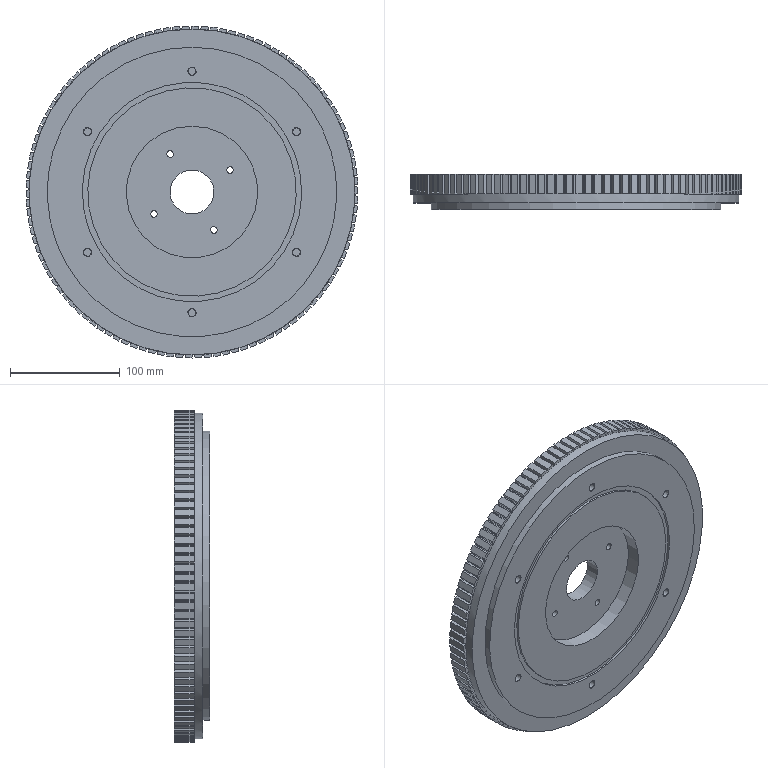Component | NX | DRIVE_SHAFT_FLYWHEEL | 1 solid | 476 faces | volume 1765684 mm3 | plane 453 | cylinder 17 | cone 6 | commonest cylinder face diameters 7 x6 6 x4 297 x1 220 x1 40 x1 120 x1 190 x1 200 x1